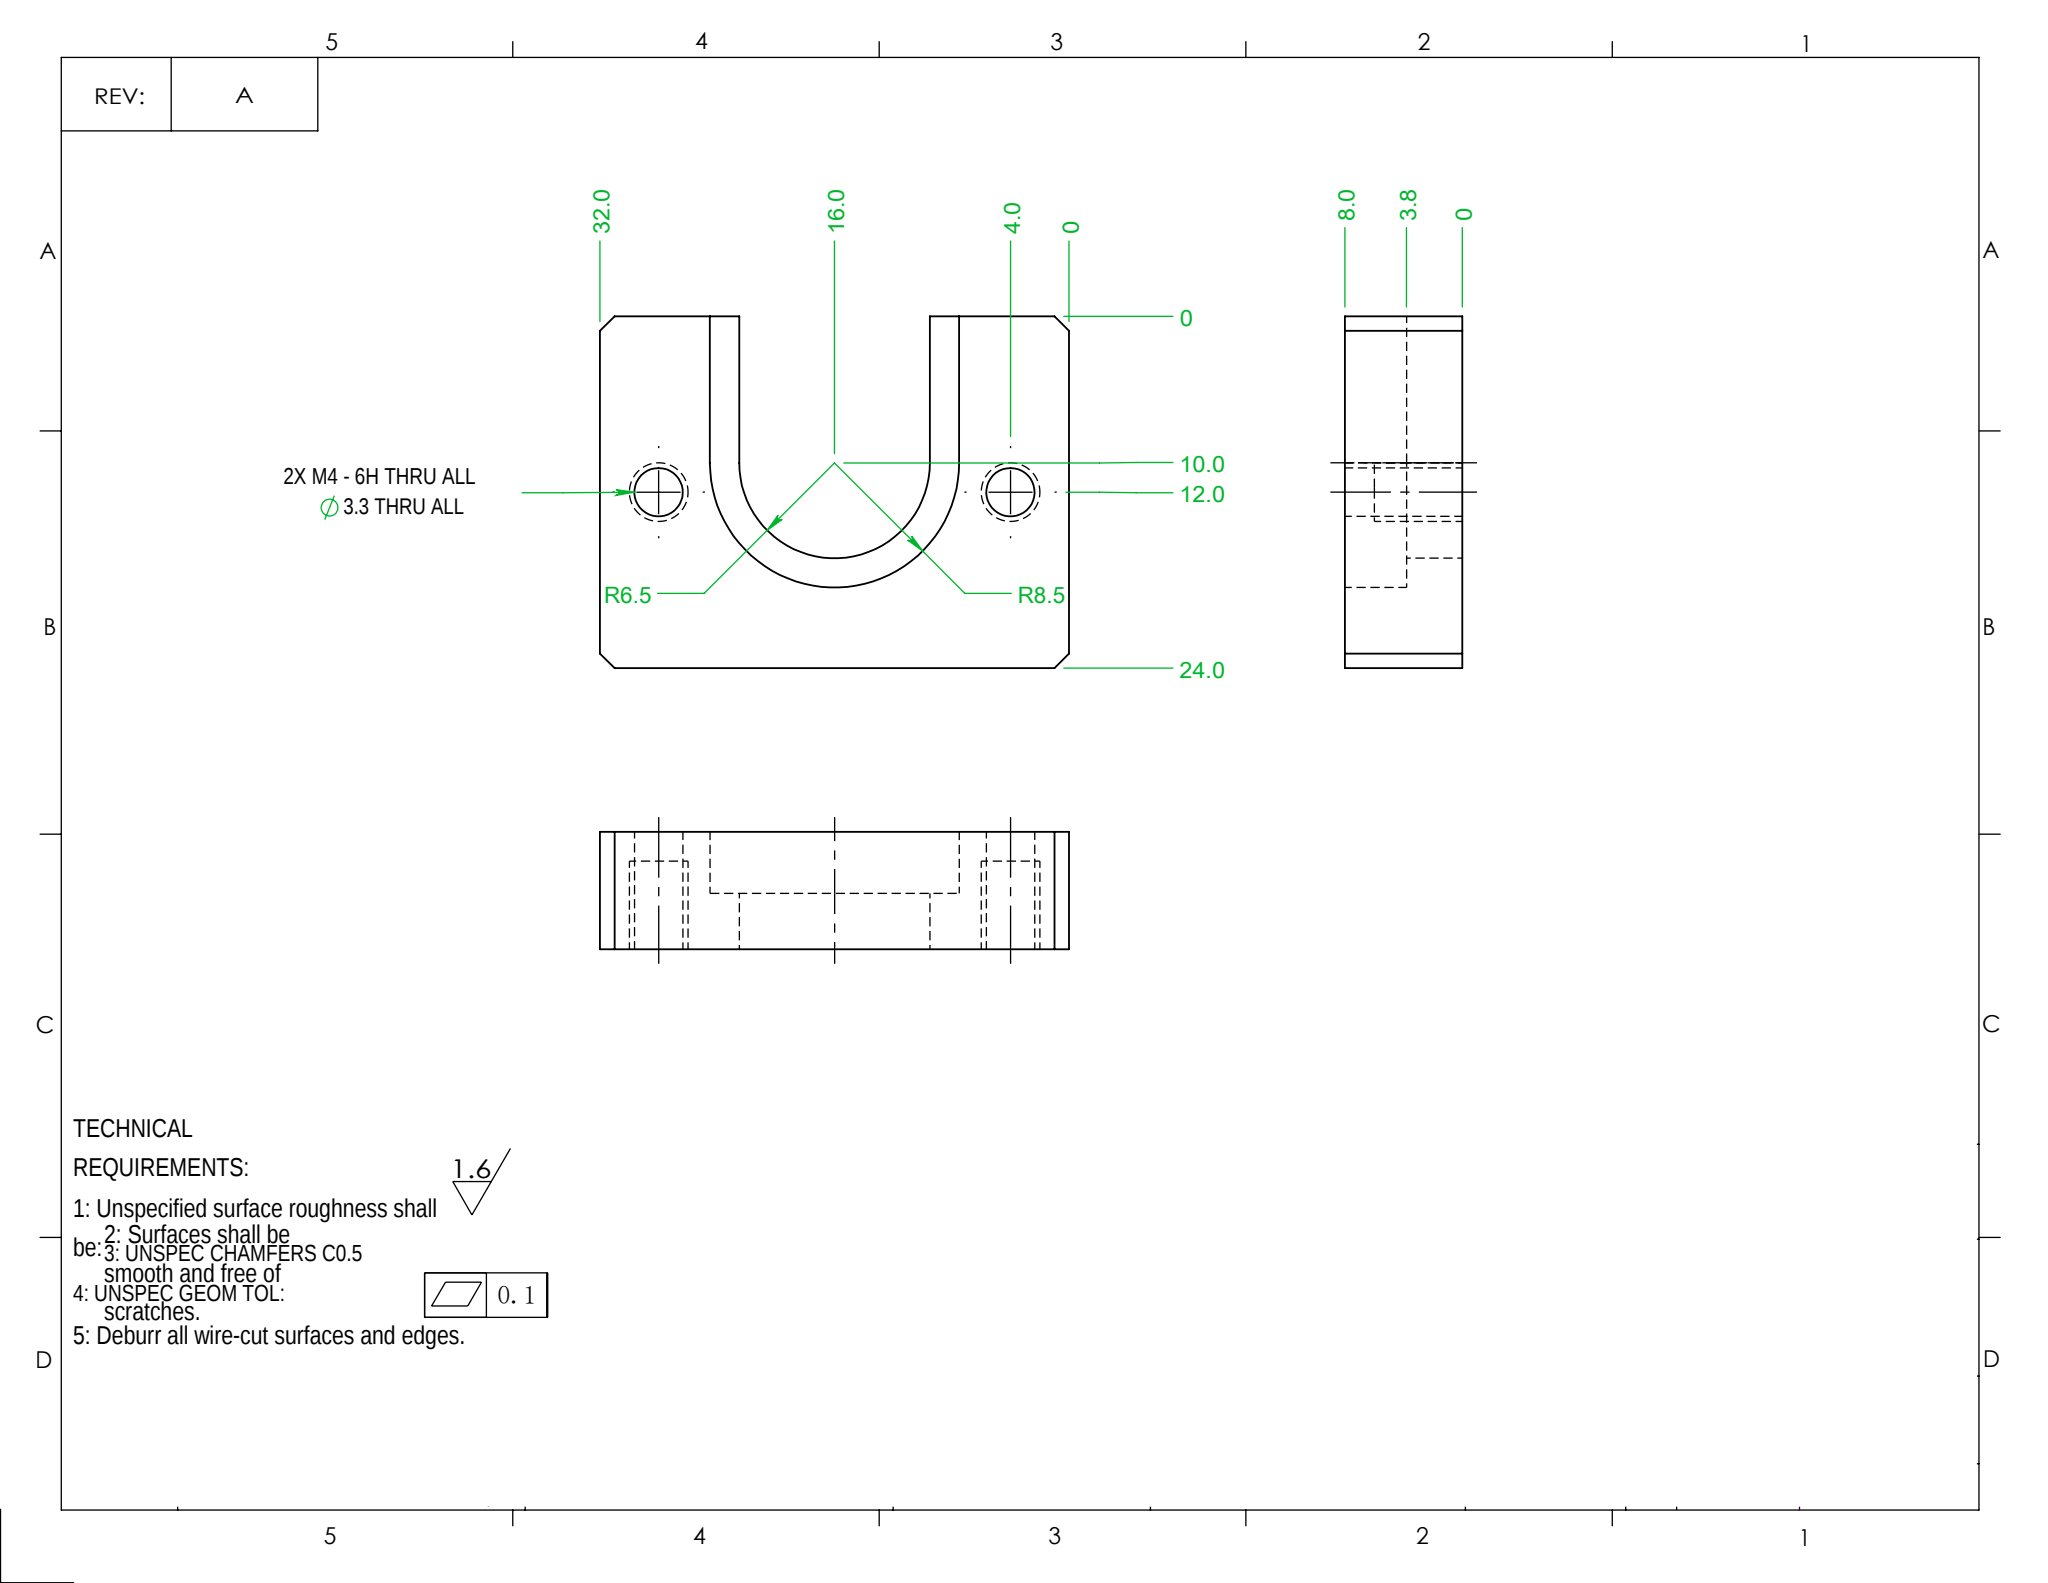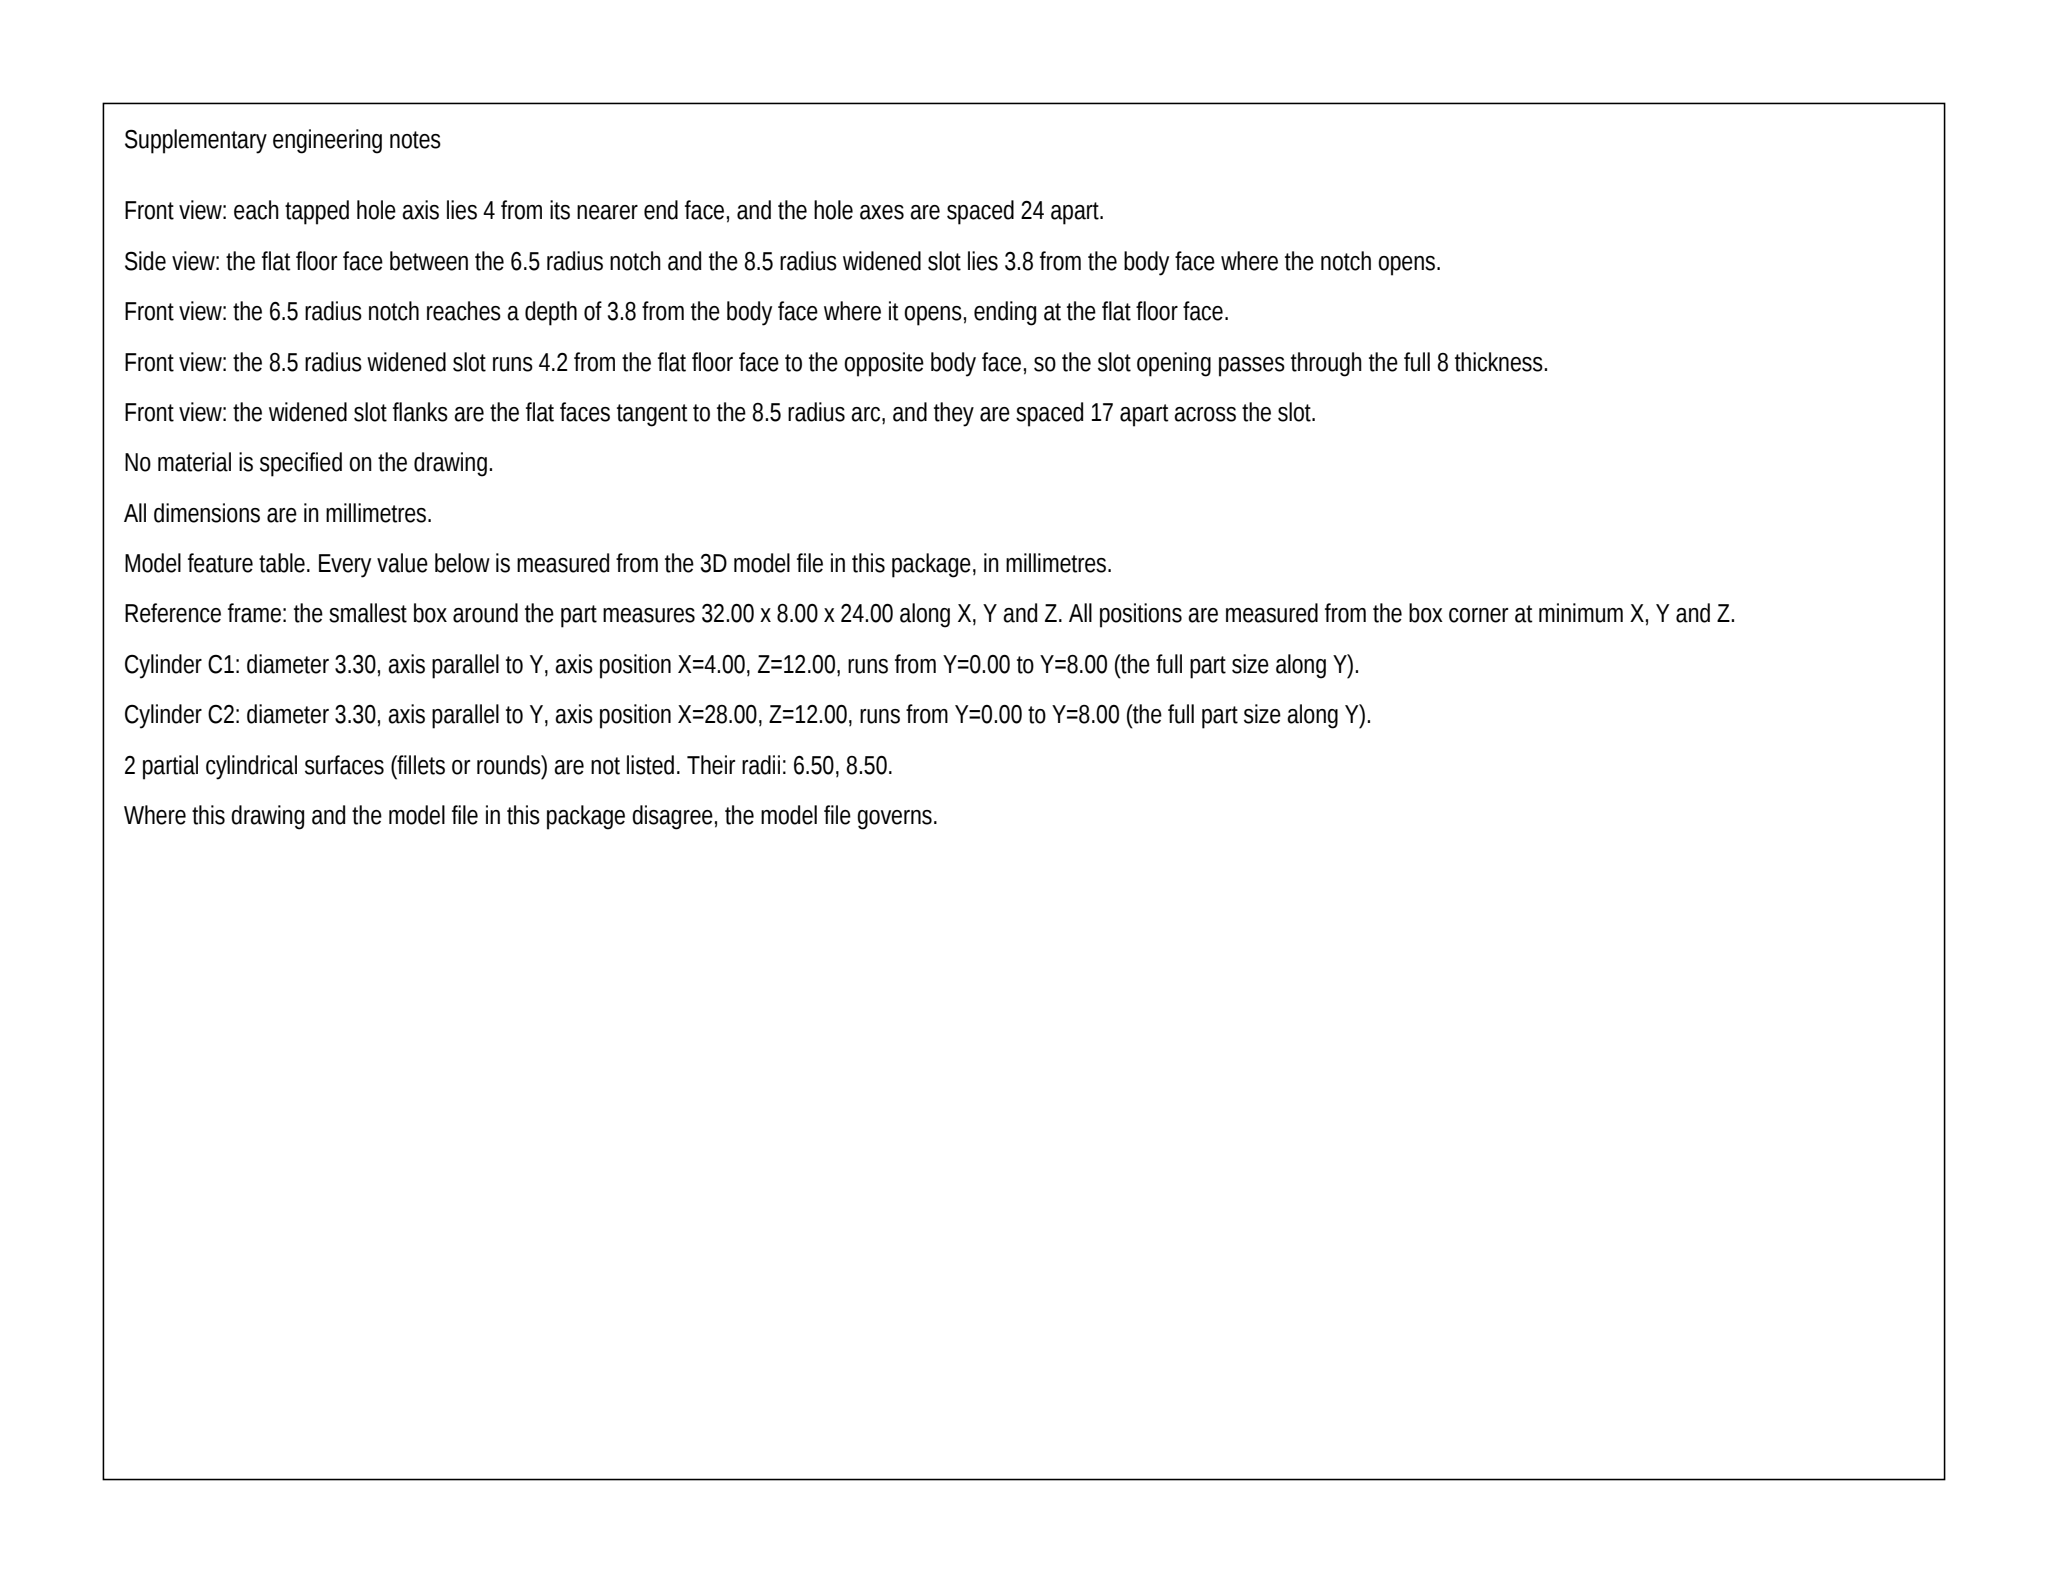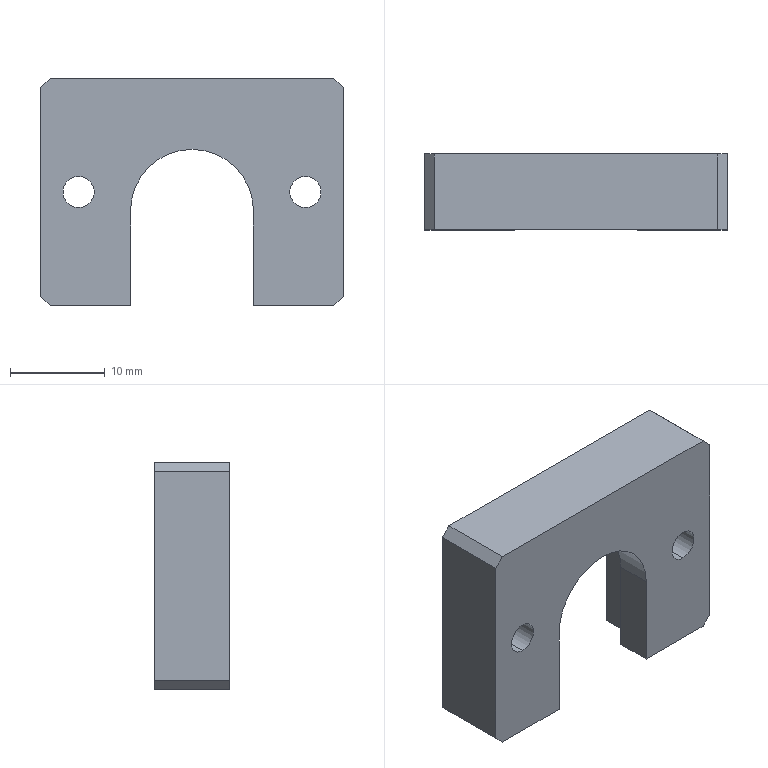Part | SolidWorks | mm | 1 solid | 24 faces | box 32 x 8 x 24 mm | volume 4054 mm3 | plane 16 | cylinder 8 | commonest cylinder face diameters 3.3 x4 13 x2 17 x2
build123d program:
from build123d import *

# Parameters (mm, degrees)
SKETCH1_W           = 32
SKETCH1_H           = 24
BOSS_EXTRUDE1_DEPTH = 8
CUT_EXTRUDE1_DEPTH  = 4.2
CUT_EXTRUDE2_DEPTH  = 41.22
CHAMFER1_SIZE       = 1
M4_TAPPED_HOLE1_D   = 3.3


with BuildPart() as part:
    # Sketch1 → Boss-Extrude1 (new body)
    with BuildSketch(Plane(origin=(0, 0, 0), x_dir=(1, 0, 0), z_dir=(0, 1, 0))):
        with Locations((16, 12)):
            Rectangle(SKETCH1_W, SKETCH1_H)
    extrude(amount=BOSS_EXTRUDE1_DEPTH)

    # Sketch2 → Cut-Extrude1 (cut)
    with BuildSketch(Plane(origin=(0, 8, 0), x_dir=(1, 0, 0), z_dir=(0, 1, 0))):
        with BuildLine():
            Line((7.5, 14), (7.5, 24))
            Line((7.5, 24), (24.5, 24))
            Line((24.5, 24), (24.5, 14))
            ThreePointArc((24.5, 14), (16, 5.5), (7.5, 14))
        make_face()
    extrude(amount=-CUT_EXTRUDE1_DEPTH, mode=Mode.SUBTRACT)

    # Sketch3 → Cut-Extrude2 (cut, through all)
    with BuildSketch(Plane(origin=(0, 3.8, 0), x_dir=(1, 0, 0), z_dir=(0, 1, 0))):
        with BuildLine():
            Line((9.5, 14), (9.5, 24))
            Line((9.5, 24), (22.5, 24))
            Line((22.5, 24), (22.5, 14))
            ThreePointArc((22.5, 14), (16, 7.5), (9.5, 14))
        make_face()
    extrude(amount=-CUT_EXTRUDE2_DEPTH, mode=Mode.SUBTRACT)

    # Chamfer1
    chamfer1_edges = [part.edges().sort_by_distance(p)[0] for p in [
        (0, 4, -24),
        (32, 4, -24),
        (32, 4, 0),
        (0, 4, 0),
    ]]
    chamfer(chamfer1_edges, length=CHAMFER1_SIZE)

    # M4 Tapped Hole1 (through all)
    with Locations(Plane(origin=(0, 0, 0), x_dir=(-1, 0, 0), z_dir=(0, -1, 0))):
        with Locations((-28, 12), (-4, 12)):
            Hole(M4_TAPPED_HOLE1_D / 2)


solid = part.part
STEP:
#1=CARTESIAN_POINT('',(28.,8.,-10.35));
#2=VERTEX_POINT('',#1);
#3=CARTESIAN_POINT('',(28.,8.,-13.65));
#4=VERTEX_POINT('',#3);
#5=CARTESIAN_POINT('',(28.,8.,-12.));
#6=DIRECTION('',(0.,-1.,0.));
#7=DIRECTION('',(0.,0.,-1.));
#8=AXIS2_PLACEMENT_3D('',#5,#6,#7);
#9=CIRCLE('',#8,1.65);
#10=EDGE_CURVE('',#2,#4,#9,.T.);
#11=ORIENTED_EDGE('',*,*,#10,.F.);
#12=CARTESIAN_POINT('',(28.,-0.,-10.35));
#13=VERTEX_POINT('',#12);
#14=CARTESIAN_POINT('',(28.,0.,-10.35));
#15=DIRECTION('',(0.,-1.,0.));
#16=VECTOR('',#15,1000.);
#17=LINE('',#14,#16);
#18=EDGE_CURVE('',#2,#13,#17,.T.);
#19=ORIENTED_EDGE('',*,*,#18,.T.);
#20=CARTESIAN_POINT('',(28.,-0.,-13.65));
#21=VERTEX_POINT('',#20);
#22=CARTESIAN_POINT('',(28.,-0.,-12.));
#23=DIRECTION('',(0.,-1.,0.));
#24=DIRECTION('',(0.,0.,-1.));
#25=AXIS2_PLACEMENT_3D('',#22,#23,#24);
#26=CIRCLE('',#25,1.65);
#27=EDGE_CURVE('',#13,#21,#26,.T.);
#28=ORIENTED_EDGE('',*,*,#27,.T.);
#29=CARTESIAN_POINT('',(28.,0.,-13.65));
#30=DIRECTION('',(0.,-1.,0.));
#31=VECTOR('',#30,1000.);
#32=LINE('',#29,#31);
#33=EDGE_CURVE('',#4,#21,#32,.T.);
#34=ORIENTED_EDGE('',*,*,#33,.F.);
#35=EDGE_LOOP('',(#11,#19,#28,#34));
#36=FACE_OUTER_BOUND('',#35,.T.);
#37=CARTESIAN_POINT('',(28.,0.,-12.));
#38=DIRECTION('',(0.,-1.,0.));
#39=DIRECTION('',(0.,0.,-1.));
#40=AXIS2_PLACEMENT_3D('',#37,#38,#39);
#41=CYLINDRICAL_SURFACE('',#40,1.65);
#42=ADVANCED_FACE('',(#36),#41,.F.);
#43=CARTESIAN_POINT('',(4.,8.,-10.35));
#44=VERTEX_POINT('',#43);
#45=CARTESIAN_POINT('',(4.,8.,-13.65));
#46=VERTEX_POINT('',#45);
#47=CARTESIAN_POINT('',(4.,8.,-12.));
#48=DIRECTION('',(0.,-1.,0.));
#49=DIRECTION('',(0.,0.,-1.));
#50=AXIS2_PLACEMENT_3D('',#47,#48,#49);
#51=CIRCLE('',#50,1.65);
#52=EDGE_CURVE('',#44,#46,#51,.T.);
#53=ORIENTED_EDGE('',*,*,#52,.F.);
#54=CARTESIAN_POINT('',(4.,-0.,-10.35));
#55=VERTEX_POINT('',#54);
#56=CARTESIAN_POINT('',(4.,0.,-10.35));
#57=DIRECTION('',(0.,-1.,0.));
#58=VECTOR('',#57,1000.);
#59=LINE('',#56,#58);
#60=EDGE_CURVE('',#44,#55,#59,.T.);
#61=ORIENTED_EDGE('',*,*,#60,.T.);
#62=CARTESIAN_POINT('',(4.,-0.,-13.65));
#63=VERTEX_POINT('',#62);
#64=CARTESIAN_POINT('',(4.,-0.,-12.));
#65=DIRECTION('',(0.,-1.,0.));
#66=DIRECTION('',(0.,0.,-1.));
#67=AXIS2_PLACEMENT_3D('',#64,#65,#66);
#68=CIRCLE('',#67,1.65);
#69=EDGE_CURVE('',#55,#63,#68,.T.);
#70=ORIENTED_EDGE('',*,*,#69,.T.);
#71=CARTESIAN_POINT('',(4.,0.,-13.65));
#72=DIRECTION('',(0.,-1.,0.));
#73=VECTOR('',#72,1000.);
#74=LINE('',#71,#73);
#75=EDGE_CURVE('',#46,#63,#74,.T.);
#76=ORIENTED_EDGE('',*,*,#75,.F.);
#77=EDGE_LOOP('',(#53,#61,#70,#76));
#78=FACE_OUTER_BOUND('',#77,.T.);
#79=CARTESIAN_POINT('',(4.,0.,-12.));
#80=DIRECTION('',(0.,-1.,0.));
#81=DIRECTION('',(0.,0.,-1.));
#82=AXIS2_PLACEMENT_3D('',#79,#80,#81);
#83=CYLINDRICAL_SURFACE('',#82,1.65);
#84=ADVANCED_FACE('',(#78),#83,.F.);
#85=CARTESIAN_POINT('',(16.,0.,-7.5));
#86=VERTEX_POINT('',#85);
#87=CARTESIAN_POINT('',(22.5,0.,-14.));
#88=VERTEX_POINT('',#87);
#89=CARTESIAN_POINT('',(16.,0.,-14.));
#90=DIRECTION('',(0.,1.,0.));
#91=DIRECTION('',(0.,0.,1.));
#92=AXIS2_PLACEMENT_3D('',#89,#90,#91);
#93=CIRCLE('',#92,6.5);
#94=EDGE_CURVE('',#86,#88,#93,.T.);
#95=ORIENTED_EDGE('',*,*,#94,.F.);
#96=CARTESIAN_POINT('',(16.,3.8,-7.5));
#97=VERTEX_POINT('',#96);
#98=CARTESIAN_POINT('',(16.,0.,-7.5));
#99=DIRECTION('',(0.,1.,0.));
#100=VECTOR('',#99,1000.);
#101=LINE('',#98,#100);
#102=EDGE_CURVE('',#86,#97,#101,.T.);
#103=ORIENTED_EDGE('',*,*,#102,.T.);
#104=CARTESIAN_POINT('',(22.5,3.8,-14.));
#105=VERTEX_POINT('',#104);
#106=CARTESIAN_POINT('',(16.,3.8,-14.));
#107=DIRECTION('',(0.,1.,0.));
#108=DIRECTION('',(0.,0.,1.));
#109=AXIS2_PLACEMENT_3D('',#106,#107,#108);
#110=CIRCLE('',#109,6.5);
#111=EDGE_CURVE('',#97,#105,#110,.T.);
#112=ORIENTED_EDGE('',*,*,#111,.T.);
#113=CARTESIAN_POINT('',(22.5,0.,-14.));
#114=DIRECTION('',(0.,1.,0.));
#115=VECTOR('',#114,1000.);
#116=LINE('',#113,#115);
#117=EDGE_CURVE('',#88,#105,#116,.T.);
#118=ORIENTED_EDGE('',*,*,#117,.F.);
#119=EDGE_LOOP('',(#95,#103,#112,#118));
#120=FACE_OUTER_BOUND('',#119,.T.);
#121=CARTESIAN_POINT('',(16.,0.,-14.));
#122=DIRECTION('',(0.,1.,0.));
#123=DIRECTION('',(0.,0.,1.));
#124=AXIS2_PLACEMENT_3D('',#121,#122,#123);
#125=CYLINDRICAL_SURFACE('',#124,6.5);
#126=ADVANCED_FACE('',(#120),#125,.F.);
#127=CARTESIAN_POINT('',(16.,3.8,-5.5));
#128=VERTEX_POINT('',#127);
#129=CARTESIAN_POINT('',(24.5,3.8,-14.));
#130=VERTEX_POINT('',#129);
#131=CARTESIAN_POINT('',(16.,3.8,-14.));
#132=DIRECTION('',(0.,1.,0.));
#133=DIRECTION('',(0.,0.,1.));
#134=AXIS2_PLACEMENT_3D('',#131,#132,#133);
#135=CIRCLE('',#134,8.5);
#136=EDGE_CURVE('',#128,#130,#135,.T.);
#137=ORIENTED_EDGE('',*,*,#136,.F.);
#138=CARTESIAN_POINT('',(16.,8.,-5.5));
#139=VERTEX_POINT('',#138);
#140=CARTESIAN_POINT('',(16.,3.8,-5.5));
#141=DIRECTION('',(0.,1.,0.));
#142=VECTOR('',#141,1000.);
#143=LINE('',#140,#142);
#144=EDGE_CURVE('',#128,#139,#143,.T.);
#145=ORIENTED_EDGE('',*,*,#144,.T.);
#146=CARTESIAN_POINT('',(24.5,8.,-14.));
#147=VERTEX_POINT('',#146);
#148=CARTESIAN_POINT('',(16.,8.,-14.));
#149=DIRECTION('',(0.,1.,0.));
#150=DIRECTION('',(0.,0.,1.));
#151=AXIS2_PLACEMENT_3D('',#148,#149,#150);
#152=CIRCLE('',#151,8.5);
#153=EDGE_CURVE('',#139,#147,#152,.T.);
#154=ORIENTED_EDGE('',*,*,#153,.T.);
#155=CARTESIAN_POINT('',(24.5,3.8,-14.));
#156=DIRECTION('',(0.,1.,0.));
#157=VECTOR('',#156,1000.);
#158=LINE('',#155,#157);
#159=EDGE_CURVE('',#130,#147,#158,.T.);
#160=ORIENTED_EDGE('',*,*,#159,.F.);
#161=EDGE_LOOP('',(#137,#145,#154,#160));
#162=FACE_OUTER_BOUND('',#161,.T.);
#163=CARTESIAN_POINT('',(16.,3.8,-14.));
#164=DIRECTION('',(0.,1.,0.));
#165=DIRECTION('',(0.,0.,1.));
#166=AXIS2_PLACEMENT_3D('',#163,#164,#165);
#167=CYLINDRICAL_SURFACE('',#166,8.5);
#168=ADVANCED_FACE('',(#162),#167,.F.);
#169=CARTESIAN_POINT('',(9.5,0.,-24.));
#170=VERTEX_POINT('',#169);
#171=CARTESIAN_POINT('',(1.,0.,-24.));
#172=VERTEX_POINT('',#171);
#173=CARTESIAN_POINT('',(0.,0.,-24.));
#174=DIRECTION('',(-1.,0.,0.));
#175=VECTOR('',#174,1000.);
#176=LINE('',#173,#175);
#177=EDGE_CURVE('',#170,#172,#176,.T.);
#178=ORIENTED_EDGE('',*,*,#177,.T.);
#179=CARTESIAN_POINT('',(1.,8.,-24.));
#180=VERTEX_POINT('',#179);
#181=CARTESIAN_POINT('',(1.,8.,-24.));
#182=DIRECTION('',(0.,1.,0.));
#183=VECTOR('',#182,1000.);
#184=LINE('',#181,#183);
#185=EDGE_CURVE('',#172,#180,#184,.T.);
#186=ORIENTED_EDGE('',*,*,#185,.T.);
#187=CARTESIAN_POINT('',(7.5,8.,-24.));
#188=VERTEX_POINT('',#187);
#189=CARTESIAN_POINT('',(0.,8.,-24.));
#190=DIRECTION('',(-1.,0.,0.));
#191=VECTOR('',#190,1000.);
#192=LINE('',#189,#191);
#193=EDGE_CURVE('',#188,#180,#192,.T.);
#194=ORIENTED_EDGE('',*,*,#193,.F.);
#195=CARTESIAN_POINT('',(7.5,3.8,-24.));
#196=VERTEX_POINT('',#195);
#197=CARTESIAN_POINT('',(7.5,3.8,-24.));
#198=DIRECTION('',(0.,1.,0.));
#199=VECTOR('',#198,1000.);
#200=LINE('',#197,#199);
#201=EDGE_CURVE('',#196,#188,#200,.T.);
#202=ORIENTED_EDGE('',*,*,#201,.F.);
#203=CARTESIAN_POINT('',(9.5,3.8,-24.));
#204=VERTEX_POINT('',#203);
#205=CARTESIAN_POINT('',(7.5,3.8,-24.));
#206=DIRECTION('',(-1.,0.,0.));
#207=VECTOR('',#206,1000.);
#208=LINE('',#205,#207);
#209=EDGE_CURVE('',#204,#196,#208,.T.);
#210=ORIENTED_EDGE('',*,*,#209,.F.);
#211=CARTESIAN_POINT('',(9.5,0.,-24.));
#212=DIRECTION('',(0.,1.,0.));
#213=VECTOR('',#212,1000.);
#214=LINE('',#211,#213);
#215=EDGE_CURVE('',#170,#204,#214,.T.);
#216=ORIENTED_EDGE('',*,*,#215,.F.);
#217=EDGE_LOOP('',(#178,#186,#194,#202,#210,#216));
#218=FACE_OUTER_BOUND('',#217,.T.);
#219=CARTESIAN_POINT('',(0.,8.,-24.));
#220=DIRECTION('',(0.,0.,1.));
#221=DIRECTION('',(1.,0.,0.));
#222=AXIS2_PLACEMENT_3D('',#219,#220,#221);
#223=PLANE('',#222);
#224=ADVANCED_FACE('',(#218),#223,.F.);
#225=CARTESIAN_POINT('',(0.,0.,-23.));
#226=VERTEX_POINT('',#225);
#227=CARTESIAN_POINT('',(0.,0.,-1.));
#228=VERTEX_POINT('',#227);
#229=CARTESIAN_POINT('',(0.,0.,0.));
#230=DIRECTION('',(-0.,0.,1.));
#231=VECTOR('',#230,1000.);
#232=LINE('',#229,#231);
#233=EDGE_CURVE('',#226,#228,#232,.T.);
#234=ORIENTED_EDGE('',*,*,#233,.T.);
#235=CARTESIAN_POINT('',(0.,8.,-1.));
#236=VERTEX_POINT('',#235);
#237=CARTESIAN_POINT('',(0.,8.,-1.));
#238=DIRECTION('',(0.,1.,0.));
#239=VECTOR('',#238,1000.);
#240=LINE('',#237,#239);
#241=EDGE_CURVE('',#228,#236,#240,.T.);
#242=ORIENTED_EDGE('',*,*,#241,.T.);
#243=CARTESIAN_POINT('',(0.,8.,-23.));
#244=VERTEX_POINT('',#243);
#245=CARTESIAN_POINT('',(0.,8.,0.));
#246=DIRECTION('',(-0.,0.,1.));
#247=VECTOR('',#246,1000.);
#248=LINE('',#245,#247);
#249=EDGE_CURVE('',#244,#236,#248,.T.);
#250=ORIENTED_EDGE('',*,*,#249,.F.);
#251=CARTESIAN_POINT('',(0.,8.,-23.));
#252=DIRECTION('',(0.,-1.,0.));
#253=VECTOR('',#252,1000.);
#254=LINE('',#251,#253);
#255=EDGE_CURVE('',#244,#226,#254,.T.);
#256=ORIENTED_EDGE('',*,*,#255,.T.);
#257=EDGE_LOOP('',(#234,#242,#250,#256));
#258=FACE_OUTER_BOUND('',#257,.T.);
#259=CARTESIAN_POINT('',(0.,8.,0.));
#260=DIRECTION('',(1.,0.,0.));
#261=DIRECTION('',(0.,0.,-1.));
#262=AXIS2_PLACEMENT_3D('',#259,#260,#261);
#263=PLANE('',#262);
#264=ADVANCED_FACE('',(#258),#263,.F.);
#265=CARTESIAN_POINT('',(1.,8.,-0.));
#266=VERTEX_POINT('',#265);
#267=CARTESIAN_POINT('',(31.,8.,-0.));
#268=VERTEX_POINT('',#267);
#269=CARTESIAN_POINT('',(0.,8.,0.));
#270=DIRECTION('',(1.,0.,0.));
#271=VECTOR('',#270,1000.);
#272=LINE('',#269,#271);
#273=EDGE_CURVE('',#266,#268,#272,.T.);
#274=ORIENTED_EDGE('',*,*,#273,.F.);
#275=CARTESIAN_POINT('',(1.,0.,-0.));
#276=VERTEX_POINT('',#275);
#277=CARTESIAN_POINT('',(1.,8.,0.));
#278=DIRECTION('',(0.,-1.,0.));
#279=VECTOR('',#278,1000.);
#280=LINE('',#277,#279);
#281=EDGE_CURVE('',#266,#276,#280,.T.);
#282=ORIENTED_EDGE('',*,*,#281,.T.);
#283=CARTESIAN_POINT('',(31.,0.,0.));
#284=VERTEX_POINT('',#283);
#285=CARTESIAN_POINT('',(0.,0.,0.));
#286=DIRECTION('',(1.,0.,0.));
#287=VECTOR('',#286,1000.);
#288=LINE('',#285,#287);
#289=EDGE_CURVE('',#276,#284,#288,.T.);
#290=ORIENTED_EDGE('',*,*,#289,.T.);
#291=CARTESIAN_POINT('',(31.,8.,0.));
#292=DIRECTION('',(0.,1.,0.));
#293=VECTOR('',#292,1000.);
#294=LINE('',#291,#293);
#295=EDGE_CURVE('',#284,#268,#294,.T.);
#296=ORIENTED_EDGE('',*,*,#295,.T.);
#297=EDGE_LOOP('',(#274,#282,#290,#296));
#298=FACE_OUTER_BOUND('',#297,.T.);
#299=CARTESIAN_POINT('',(0.,8.,0.));
#300=DIRECTION('',(0.,0.,-1.));
#301=DIRECTION('',(-1.,0.,0.));
#302=AXIS2_PLACEMENT_3D('',#299,#300,#301);
#303=PLANE('',#302);
#304=ADVANCED_FACE('',(#298),#303,.F.);
#305=CARTESIAN_POINT('',(32.,8.,-1.));
#306=VERTEX_POINT('',#305);
#307=CARTESIAN_POINT('',(32.,8.,-23.));
#308=VERTEX_POINT('',#307);
#309=CARTESIAN_POINT('',(32.,8.,0.));
#310=DIRECTION('',(-0.,0.,-1.));
#311=VECTOR('',#310,1000.);
#312=LINE('',#309,#311);
#313=EDGE_CURVE('',#306,#308,#312,.T.);
#314=ORIENTED_EDGE('',*,*,#313,.F.);
#315=CARTESIAN_POINT('',(32.,0.,-1.));
#316=VERTEX_POINT('',#315);
#317=CARTESIAN_POINT('',(32.,8.,-1.));
#318=DIRECTION('',(0.,-1.,0.));
#319=VECTOR('',#318,1000.);
#320=LINE('',#317,#319);
#321=EDGE_CURVE('',#306,#316,#320,.T.);
#322=ORIENTED_EDGE('',*,*,#321,.T.);
#323=CARTESIAN_POINT('',(32.,0.,-23.));
#324=VERTEX_POINT('',#323);
#325=CARTESIAN_POINT('',(32.,0.,0.));
#326=DIRECTION('',(-0.,0.,-1.));
#327=VECTOR('',#326,1000.);
#328=LINE('',#325,#327);
#329=EDGE_CURVE('',#316,#324,#328,.T.);
#330=ORIENTED_EDGE('',*,*,#329,.T.);
#331=CARTESIAN_POINT('',(32.,8.,-23.));
#332=DIRECTION('',(0.,1.,0.));
#333=VECTOR('',#332,1000.);
#334=LINE('',#331,#333);
#335=EDGE_CURVE('',#324,#308,#334,.T.);
#336=ORIENTED_EDGE('',*,*,#335,.T.);
#337=EDGE_LOOP('',(#314,#322,#330,#336));
#338=FACE_OUTER_BOUND('',#337,.T.);
#339=CARTESIAN_POINT('',(32.,8.,0.));
#340=DIRECTION('',(-1.,0.,0.));
#341=DIRECTION('',(0.,0.,1.));
#342=AXIS2_PLACEMENT_3D('',#339,#340,#341);
#343=PLANE('',#342);
#344=ADVANCED_FACE('',(#338),#343,.F.);
#345=CARTESIAN_POINT('',(31.,8.,-24.));
#346=VERTEX_POINT('',#345);
#347=CARTESIAN_POINT('',(24.5,8.,-24.));
#348=VERTEX_POINT('',#347);
#349=CARTESIAN_POINT('',(0.,8.,-24.));
#350=DIRECTION('',(-1.,0.,0.));
#351=VECTOR('',#350,1000.);
#352=LINE('',#349,#351);
#353=EDGE_CURVE('',#346,#348,#352,.T.);
#354=ORIENTED_EDGE('',*,*,#353,.F.);
#355=CARTESIAN_POINT('',(31.,0.,-24.));
#356=VERTEX_POINT('',#355);
#357=CARTESIAN_POINT('',(31.,8.,-24.));
#358=DIRECTION('',(0.,-1.,0.));
#359=VECTOR('',#358,1000.);
#360=LINE('',#357,#359);
#361=EDGE_CURVE('',#346,#356,#360,.T.);
#362=ORIENTED_EDGE('',*,*,#361,.T.);
#363=CARTESIAN_POINT('',(22.5,0.,-24.));
#364=VERTEX_POINT('',#363);
#365=CARTESIAN_POINT('',(0.,0.,-24.));
#366=DIRECTION('',(-1.,0.,0.));
#367=VECTOR('',#366,1000.);
#368=LINE('',#365,#367);
#369=EDGE_CURVE('',#356,#364,#368,.T.);
#370=ORIENTED_EDGE('',*,*,#369,.T.);
#371=CARTESIAN_POINT('',(22.5,3.8,-24.));
#372=VERTEX_POINT('',#371);
#373=CARTESIAN_POINT('',(22.5,0.,-24.));
#374=DIRECTION('',(0.,1.,0.));
#375=VECTOR('',#374,1000.);
#376=LINE('',#373,#375);
#377=EDGE_CURVE('',#364,#372,#376,.T.);
#378=ORIENTED_EDGE('',*,*,#377,.T.);
#379=CARTESIAN_POINT('',(24.5,3.8,-24.));
#380=VERTEX_POINT('',#379);
#381=CARTESIAN_POINT('',(7.5,3.8,-24.));
#382=DIRECTION('',(-1.,0.,0.));
#383=VECTOR('',#382,1000.);
#384=LINE('',#381,#383);
#385=EDGE_CURVE('',#380,#372,#384,.T.);
#386=ORIENTED_EDGE('',*,*,#385,.F.);
#387=CARTESIAN_POINT('',(24.5,3.8,-24.));
#388=DIRECTION('',(0.,1.,0.));
#389=VECTOR('',#388,1000.);
#390=LINE('',#387,#389);
#391=EDGE_CURVE('',#380,#348,#390,.T.);
#392=ORIENTED_EDGE('',*,*,#391,.T.);
#393=EDGE_LOOP('',(#354,#362,#370,#378,#386,#392));
#394=FACE_OUTER_BOUND('',#393,.T.);
#395=CARTESIAN_POINT('',(0.,8.,-24.));
#396=DIRECTION('',(0.,0.,1.));
#397=DIRECTION('',(1.,0.,0.));
#398=AXIS2_PLACEMENT_3D('',#395,#396,#397);
#399=PLANE('',#398);
#400=ADVANCED_FACE('',(#394),#399,.F.);
#401=CARTESIAN_POINT('',(28.,8.,-12.));
#402=DIRECTION('',(0.,-1.,0.));
#403=DIRECTION('',(0.,0.,-1.));
#404=AXIS2_PLACEMENT_3D('',#401,#402,#403);
#405=CIRCLE('',#404,1.65);
#406=EDGE_CURVE('',#4,#2,#405,.T.);
#407=ORIENTED_EDGE('',*,*,#406,.T.);
#408=ORIENTED_EDGE('',*,*,#10,.T.);
#409=EDGE_LOOP('',(#407,#408));
#410=FACE_BOUND('',#409,.T.);
#411=CARTESIAN_POINT('',(4.,8.,-12.));
#412=DIRECTION('',(0.,-1.,0.));
#413=DIRECTION('',(0.,0.,-1.));
#414=AXIS2_PLACEMENT_3D('',#411,#412,#413);
#415=CIRCLE('',#414,1.65);
#416=EDGE_CURVE('',#46,#44,#415,.T.);
#417=ORIENTED_EDGE('',*,*,#416,.T.);
#418=ORIENTED_EDGE('',*,*,#52,.T.);
#419=EDGE_LOOP('',(#417,#418));
#420=FACE_BOUND('',#419,.T.);
#421=ORIENTED_EDGE('',*,*,#249,.T.);
#422=CARTESIAN_POINT('',(1.,8.,0.));
#423=DIRECTION('',(0.7071,0.,0.7071));
#424=VECTOR('',#423,1000.);
#425=LINE('',#422,#424);
#426=EDGE_CURVE('',#236,#266,#425,.T.);
#427=ORIENTED_EDGE('',*,*,#426,.T.);
#428=ORIENTED_EDGE('',*,*,#273,.T.);
#429=CARTESIAN_POINT('',(32.,8.,-1.));
#430=DIRECTION('',(0.7071,0.,-0.7071));
#431=VECTOR('',#430,1000.);
#432=LINE('',#429,#431);
#433=EDGE_CURVE('',#268,#306,#432,.T.);
#434=ORIENTED_EDGE('',*,*,#433,.T.);
#435=ORIENTED_EDGE('',*,*,#313,.T.);
#436=CARTESIAN_POINT('',(31.,8.,-24.));
#437=DIRECTION('',(-0.7071,0.,-0.7071));
#438=VECTOR('',#437,1000.);
#439=LINE('',#436,#438);
#440=EDGE_CURVE('',#308,#346,#439,.T.);
#441=ORIENTED_EDGE('',*,*,#440,.T.);
#442=ORIENTED_EDGE('',*,*,#353,.T.);
#443=CARTESIAN_POINT('',(24.5,8.,-24.));
#444=DIRECTION('',(0.,0.,-1.));
#445=VECTOR('',#444,1000.);
#446=LINE('',#443,#445);
#447=EDGE_CURVE('',#147,#348,#446,.T.);
#448=ORIENTED_EDGE('',*,*,#447,.F.);
#449=ORIENTED_EDGE('',*,*,#153,.F.);
#450=CARTESIAN_POINT('',(7.5,8.,-14.));
#451=VERTEX_POINT('',#450);
#452=CARTESIAN_POINT('',(16.,8.,-14.));
#453=DIRECTION('',(0.,1.,0.));
#454=DIRECTION('',(0.,0.,1.));
#455=AXIS2_PLACEMENT_3D('',#452,#453,#454);
#456=CIRCLE('',#455,8.5);
#457=EDGE_CURVE('',#451,#139,#456,.T.);
#458=ORIENTED_EDGE('',*,*,#457,.F.);
#459=CARTESIAN_POINT('',(7.5,8.,-14.));
#460=DIRECTION('',(0.,0.,1.));
#461=VECTOR('',#460,1000.);
#462=LINE('',#459,#461);
#463=EDGE_CURVE('',#188,#451,#462,.T.);
#464=ORIENTED_EDGE('',*,*,#463,.F.);
#465=ORIENTED_EDGE('',*,*,#193,.T.);
#466=CARTESIAN_POINT('',(0.,8.,-23.));
#467=DIRECTION('',(-0.7071,0.,0.7071));
#468=VECTOR('',#467,1000.);
#469=LINE('',#466,#468);
#470=EDGE_CURVE('',#180,#244,#469,.T.);
#471=ORIENTED_EDGE('',*,*,#470,.T.);
#472=EDGE_LOOP('',(#421,#427,#428,#434,#435,#441,#442,#448,#449,#458,#464,#465,#471));
#473=FACE_OUTER_BOUND('',#472,.T.);
#474=CARTESIAN_POINT('',(0.,8.,0.));
#475=DIRECTION('',(0.,-1.,0.));
#476=DIRECTION('',(0.,0.,-1.));
#477=AXIS2_PLACEMENT_3D('',#474,#475,#476);
#478=PLANE('',#477);
#479=ADVANCED_FACE('',(#410,#420,#473),#478,.F.);
#480=CARTESIAN_POINT('',(28.,-0.,-12.));
#481=DIRECTION('',(0.,-1.,0.));
#482=DIRECTION('',(0.,0.,-1.));
#483=AXIS2_PLACEMENT_3D('',#480,#481,#482);
#484=CIRCLE('',#483,1.65);
#485=EDGE_CURVE('',#21,#13,#484,.T.);
#486=ORIENTED_EDGE('',*,*,#485,.F.);
#487=ORIENTED_EDGE('',*,*,#27,.F.);
#488=EDGE_LOOP('',(#486,#487));
#489=FACE_BOUND('',#488,.T.);
#490=CARTESIAN_POINT('',(4.,-0.,-12.));
#491=DIRECTION('',(0.,-1.,0.));
#492=DIRECTION('',(0.,0.,-1.));
#493=AXIS2_PLACEMENT_3D('',#490,#491,#492);
#494=CIRCLE('',#493,1.65);
#495=EDGE_CURVE('',#63,#55,#494,.T.);
#496=ORIENTED_EDGE('',*,*,#495,.F.);
#497=ORIENTED_EDGE('',*,*,#69,.F.);
#498=EDGE_LOOP('',(#496,#497));
#499=FACE_BOUND('',#498,.T.);
#500=ORIENTED_EDGE('',*,*,#289,.F.);
#501=CARTESIAN_POINT('',(0.5,0.,-0.5));
#502=DIRECTION('',(-0.7071,0.,-0.7071));
#503=VECTOR('',#502,1000.);
#504=LINE('',#501,#503);
#505=EDGE_CURVE('',#276,#228,#504,.T.);
#506=ORIENTED_EDGE('',*,*,#505,.T.);
#507=ORIENTED_EDGE('',*,*,#233,.F.);
#508=CARTESIAN_POINT('',(-11.5,0.,-11.5));
#509=DIRECTION('',(0.7071,0.,-0.7071));
#510=VECTOR('',#509,1000.);
#511=LINE('',#508,#510);
#512=EDGE_CURVE('',#226,#172,#511,.T.);
#513=ORIENTED_EDGE('',*,*,#512,.T.);
#514=ORIENTED_EDGE('',*,*,#177,.F.);
#515=CARTESIAN_POINT('',(9.5,0.,-14.));
#516=VERTEX_POINT('',#515);
#517=CARTESIAN_POINT('',(9.5,0.,-14.));
#518=DIRECTION('',(0.,0.,1.));
#519=VECTOR('',#518,1000.);
#520=LINE('',#517,#519);
#521=EDGE_CURVE('',#170,#516,#520,.T.);
#522=ORIENTED_EDGE('',*,*,#521,.T.);
#523=CARTESIAN_POINT('',(16.,0.,-14.));
#524=DIRECTION('',(0.,1.,0.));
#525=DIRECTION('',(0.,0.,1.));
#526=AXIS2_PLACEMENT_3D('',#523,#524,#525);
#527=CIRCLE('',#526,6.5);
#528=EDGE_CURVE('',#516,#86,#527,.T.);
#529=ORIENTED_EDGE('',*,*,#528,.T.);
#530=ORIENTED_EDGE('',*,*,#94,.T.);
#531=CARTESIAN_POINT('',(22.5,0.,-24.));
#532=DIRECTION('',(0.,0.,-1.));
#533=VECTOR('',#532,1000.);
#534=LINE('',#531,#533);
#535=EDGE_CURVE('',#88,#364,#534,.T.);
#536=ORIENTED_EDGE('',*,*,#535,.T.);
#537=ORIENTED_EDGE('',*,*,#369,.F.);
#538=CARTESIAN_POINT('',(27.5,0.,-27.5));
#539=DIRECTION('',(0.7071,0.,0.7071));
#540=VECTOR('',#539,1000.);
#541=LINE('',#538,#540);
#542=EDGE_CURVE('',#356,#324,#541,.T.);
#543=ORIENTED_EDGE('',*,*,#542,.T.);
#544=ORIENTED_EDGE('',*,*,#329,.F.);
#545=CARTESIAN_POINT('',(15.5,0.,15.5));
#546=DIRECTION('',(-0.7071,0.,0.7071));
#547=VECTOR('',#546,1000.);
#548=LINE('',#545,#547);
#549=EDGE_CURVE('',#316,#284,#548,.T.);
#550=ORIENTED_EDGE('',*,*,#549,.T.);
#551=EDGE_LOOP('',(#500,#506,#507,#513,#514,#522,#529,#530,#536,#537,#543,#544,#550));
#552=FACE_OUTER_BOUND('',#551,.T.);
#553=CARTESIAN_POINT('',(0.,0.,0.));
#554=DIRECTION('',(0.,-1.,0.));
#555=DIRECTION('',(0.,0.,-1.));
#556=AXIS2_PLACEMENT_3D('',#553,#554,#555);
#557=PLANE('',#556);
#558=ADVANCED_FACE('',(#489,#499,#552),#557,.T.);
#559=ORIENTED_EDGE('',*,*,#144,.F.);
#560=CARTESIAN_POINT('',(7.5,3.8,-14.));
#561=VERTEX_POINT('',#560);
#562=CARTESIAN_POINT('',(16.,3.8,-14.));
#563=DIRECTION('',(0.,1.,0.));
#564=DIRECTION('',(0.,0.,1.));
#565=AXIS2_PLACEMENT_3D('',#562,#563,#564);
#566=CIRCLE('',#565,8.5);
#567=EDGE_CURVE('',#561,#128,#566,.T.);
#568=ORIENTED_EDGE('',*,*,#567,.F.);
#569=CARTESIAN_POINT('',(7.5,3.8,-14.));
#570=DIRECTION('',(0.,1.,0.));
#571=VECTOR('',#570,1000.);
#572=LINE('',#569,#571);
#573=EDGE_CURVE('',#561,#451,#572,.T.);
#574=ORIENTED_EDGE('',*,*,#573,.T.);
#575=ORIENTED_EDGE('',*,*,#457,.T.);
#576=EDGE_LOOP('',(#559,#568,#574,#575));
#577=FACE_OUTER_BOUND('',#576,.T.);
#578=CARTESIAN_POINT('',(16.,3.8,-14.));
#579=DIRECTION('',(0.,1.,0.));
#580=DIRECTION('',(0.,0.,1.));
#581=AXIS2_PLACEMENT_3D('',#578,#579,#580);
#582=CYLINDRICAL_SURFACE('',#581,8.5);
#583=ADVANCED_FACE('',(#577),#582,.F.);
#584=ORIENTED_EDGE('',*,*,#463,.T.);
#585=ORIENTED_EDGE('',*,*,#573,.F.);
#586=CARTESIAN_POINT('',(7.5,3.8,-14.));
#587=DIRECTION('',(0.,0.,1.));
#588=VECTOR('',#587,1000.);
#589=LINE('',#586,#588);
#590=EDGE_CURVE('',#196,#561,#589,.T.);
#591=ORIENTED_EDGE('',*,*,#590,.F.);
#592=ORIENTED_EDGE('',*,*,#201,.T.);
#593=EDGE_LOOP('',(#584,#585,#591,#592));
#594=FACE_OUTER_BOUND('',#593,.T.);
#595=CARTESIAN_POINT('',(7.5,3.8,-14.));
#596=DIRECTION('',(-1.,0.,0.));
#597=DIRECTION('',(0.,0.,1.));
#598=AXIS2_PLACEMENT_3D('',#595,#596,#597);
#599=PLANE('',#598);
#600=ADVANCED_FACE('',(#594),#599,.F.);
#601=ORIENTED_EDGE('',*,*,#447,.T.);
#602=ORIENTED_EDGE('',*,*,#391,.F.);
#603=CARTESIAN_POINT('',(24.5,3.8,-24.));
#604=DIRECTION('',(0.,0.,-1.));
#605=VECTOR('',#604,1000.);
#606=LINE('',#603,#605);
#607=EDGE_CURVE('',#130,#380,#606,.T.);
#608=ORIENTED_EDGE('',*,*,#607,.F.);
#609=ORIENTED_EDGE('',*,*,#159,.T.);
#610=EDGE_LOOP('',(#601,#602,#608,#609));
#611=FACE_OUTER_BOUND('',#610,.T.);
#612=CARTESIAN_POINT('',(24.5,3.8,-24.));
#613=DIRECTION('',(1.,0.,0.));
#614=DIRECTION('',(0.,0.,-1.));
#615=AXIS2_PLACEMENT_3D('',#612,#613,#614);
#616=PLANE('',#615);
#617=ADVANCED_FACE('',(#611),#616,.F.);
#618=CARTESIAN_POINT('',(9.5,3.8,-14.));
#619=VERTEX_POINT('',#618);
#620=CARTESIAN_POINT('',(9.5,3.8,-14.));
#621=DIRECTION('',(0.,0.,1.));
#622=VECTOR('',#621,1000.);
#623=LINE('',#620,#622);
#624=EDGE_CURVE('',#204,#619,#623,.T.);
#625=ORIENTED_EDGE('',*,*,#624,.F.);
#626=ORIENTED_EDGE('',*,*,#209,.T.);
#627=ORIENTED_EDGE('',*,*,#590,.T.);
#628=ORIENTED_EDGE('',*,*,#567,.T.);
#629=ORIENTED_EDGE('',*,*,#136,.T.);
#630=ORIENTED_EDGE('',*,*,#607,.T.);
#631=ORIENTED_EDGE('',*,*,#385,.T.);
#632=CARTESIAN_POINT('',(22.5,3.8,-24.));
#633=DIRECTION('',(0.,0.,-1.));
#634=VECTOR('',#633,1000.);
#635=LINE('',#632,#634);
#636=EDGE_CURVE('',#105,#372,#635,.T.);
#637=ORIENTED_EDGE('',*,*,#636,.F.);
#638=ORIENTED_EDGE('',*,*,#111,.F.);
#639=CARTESIAN_POINT('',(16.,3.8,-14.));
#640=DIRECTION('',(0.,1.,0.));
#641=DIRECTION('',(0.,0.,1.));
#642=AXIS2_PLACEMENT_3D('',#639,#640,#641);
#643=CIRCLE('',#642,6.5);
#644=EDGE_CURVE('',#619,#97,#643,.T.);
#645=ORIENTED_EDGE('',*,*,#644,.F.);
#646=EDGE_LOOP('',(#625,#626,#627,#628,#629,#630,#631,#637,#638,#645));
#647=FACE_OUTER_BOUND('',#646,.T.);
#648=CARTESIAN_POINT('',(16.,3.8,-14.));
#649=DIRECTION('',(0.,1.,0.));
#650=DIRECTION('',(0.,0.,1.));
#651=AXIS2_PLACEMENT_3D('',#648,#649,#650);
#652=PLANE('',#651);
#653=ADVANCED_FACE('',(#647),#652,.T.);
#654=ORIENTED_EDGE('',*,*,#102,.F.);
#655=ORIENTED_EDGE('',*,*,#528,.F.);
#656=CARTESIAN_POINT('',(9.5,0.,-14.));
#657=DIRECTION('',(0.,1.,0.));
#658=VECTOR('',#657,1000.);
#659=LINE('',#656,#658);
#660=EDGE_CURVE('',#516,#619,#659,.T.);
#661=ORIENTED_EDGE('',*,*,#660,.T.);
#662=ORIENTED_EDGE('',*,*,#644,.T.);
#663=EDGE_LOOP('',(#654,#655,#661,#662));
#664=FACE_OUTER_BOUND('',#663,.T.);
#665=CARTESIAN_POINT('',(16.,0.,-14.));
#666=DIRECTION('',(0.,1.,0.));
#667=DIRECTION('',(0.,0.,1.));
#668=AXIS2_PLACEMENT_3D('',#665,#666,#667);
#669=CYLINDRICAL_SURFACE('',#668,6.5);
#670=ADVANCED_FACE('',(#664),#669,.F.);
#671=ORIENTED_EDGE('',*,*,#624,.T.);
#672=ORIENTED_EDGE('',*,*,#660,.F.);
#673=ORIENTED_EDGE('',*,*,#521,.F.);
#674=ORIENTED_EDGE('',*,*,#215,.T.);
#675=EDGE_LOOP('',(#671,#672,#673,#674));
#676=FACE_OUTER_BOUND('',#675,.T.);
#677=CARTESIAN_POINT('',(9.5,0.,-14.));
#678=DIRECTION('',(-1.,0.,0.));
#679=DIRECTION('',(0.,0.,1.));
#680=AXIS2_PLACEMENT_3D('',#677,#678,#679);
#681=PLANE('',#680);
#682=ADVANCED_FACE('',(#676),#681,.F.);
#683=ORIENTED_EDGE('',*,*,#636,.T.);
#684=ORIENTED_EDGE('',*,*,#377,.F.);
#685=ORIENTED_EDGE('',*,*,#535,.F.);
#686=ORIENTED_EDGE('',*,*,#117,.T.);
#687=EDGE_LOOP('',(#683,#684,#685,#686));
#688=FACE_OUTER_BOUND('',#687,.T.);
#689=CARTESIAN_POINT('',(22.5,0.,-24.));
#690=DIRECTION('',(1.,0.,0.));
#691=DIRECTION('',(0.,0.,-1.));
#692=AXIS2_PLACEMENT_3D('',#689,#690,#691);
#693=PLANE('',#692);
#694=ADVANCED_FACE('',(#688),#693,.F.);
#695=ORIENTED_EDGE('',*,*,#426,.F.);
#696=ORIENTED_EDGE('',*,*,#241,.F.);
#697=ORIENTED_EDGE('',*,*,#505,.F.);
#698=ORIENTED_EDGE('',*,*,#281,.F.);
#699=EDGE_LOOP('',(#695,#696,#697,#698));
#700=FACE_OUTER_BOUND('',#699,.T.);
#701=CARTESIAN_POINT('',(1.,8.,0.));
#702=DIRECTION('',(0.7071,0.,-0.7071));
#703=DIRECTION('',(0.,-1.,0.));
#704=AXIS2_PLACEMENT_3D('',#701,#702,#703);
#705=PLANE('',#704);
#706=ADVANCED_FACE('',(#700),#705,.F.);
#707=ORIENTED_EDGE('',*,*,#433,.F.);
#708=ORIENTED_EDGE('',*,*,#295,.F.);
#709=ORIENTED_EDGE('',*,*,#549,.F.);
#710=ORIENTED_EDGE('',*,*,#321,.F.);
#711=EDGE_LOOP('',(#707,#708,#709,#710));
#712=FACE_OUTER_BOUND('',#711,.T.);
#713=CARTESIAN_POINT('',(32.,8.,-1.));
#714=DIRECTION('',(-0.7071,0.,-0.7071));
#715=DIRECTION('',(0.,-1.,0.));
#716=AXIS2_PLACEMENT_3D('',#713,#714,#715);
#717=PLANE('',#716);
#718=ADVANCED_FACE('',(#712),#717,.F.);
#719=ORIENTED_EDGE('',*,*,#470,.F.);
#720=ORIENTED_EDGE('',*,*,#185,.F.);
#721=ORIENTED_EDGE('',*,*,#512,.F.);
#722=ORIENTED_EDGE('',*,*,#255,.F.);
#723=EDGE_LOOP('',(#719,#720,#721,#722));
#724=FACE_OUTER_BOUND('',#723,.T.);
#725=CARTESIAN_POINT('',(0.,8.,-23.));
#726=DIRECTION('',(0.7071,0.,0.7071));
#727=DIRECTION('',(0.,-1.,0.));
#728=AXIS2_PLACEMENT_3D('',#725,#726,#727);
#729=PLANE('',#728);
#730=ADVANCED_FACE('',(#724),#729,.F.);
#731=ORIENTED_EDGE('',*,*,#440,.F.);
#732=ORIENTED_EDGE('',*,*,#335,.F.);
#733=ORIENTED_EDGE('',*,*,#542,.F.);
#734=ORIENTED_EDGE('',*,*,#361,.F.);
#735=EDGE_LOOP('',(#731,#732,#733,#734));
#736=FACE_OUTER_BOUND('',#735,.T.);
#737=CARTESIAN_POINT('',(31.,8.,-24.));
#738=DIRECTION('',(-0.7071,0.,0.7071));
#739=DIRECTION('',(0.,-1.,0.));
#740=AXIS2_PLACEMENT_3D('',#737,#738,#739);
#741=PLANE('',#740);
#742=ADVANCED_FACE('',(#736),#741,.F.);
#743=ORIENTED_EDGE('',*,*,#60,.F.);
#744=ORIENTED_EDGE('',*,*,#416,.F.);
#745=ORIENTED_EDGE('',*,*,#75,.T.);
#746=ORIENTED_EDGE('',*,*,#495,.T.);
#747=EDGE_LOOP('',(#743,#744,#745,#746));
#748=FACE_OUTER_BOUND('',#747,.T.);
#749=CARTESIAN_POINT('',(4.,0.,-12.));
#750=DIRECTION('',(0.,-1.,0.));
#751=DIRECTION('',(0.,0.,-1.));
#752=AXIS2_PLACEMENT_3D('',#749,#750,#751);
#753=CYLINDRICAL_SURFACE('',#752,1.65);
#754=ADVANCED_FACE('',(#748),#753,.F.);
#755=ORIENTED_EDGE('',*,*,#18,.F.);
#756=ORIENTED_EDGE('',*,*,#406,.F.);
#757=ORIENTED_EDGE('',*,*,#33,.T.);
#758=ORIENTED_EDGE('',*,*,#485,.T.);
#759=EDGE_LOOP('',(#755,#756,#757,#758));
#760=FACE_OUTER_BOUND('',#759,.T.);
#761=CARTESIAN_POINT('',(28.,0.,-12.));
#762=DIRECTION('',(0.,-1.,0.));
#763=DIRECTION('',(0.,0.,-1.));
#764=AXIS2_PLACEMENT_3D('',#761,#762,#763);
#765=CYLINDRICAL_SURFACE('',#764,1.65);
#766=ADVANCED_FACE('',(#760),#765,.F.);
#767=CLOSED_SHELL('',(#42,#84,#126,#168,#224,#264,#304,#344,#400,#479,#558,#583,#600,#617,#653,#670,#682,#694,#706,#718,#730,#742,#754,#766));
#768=MANIFOLD_SOLID_BREP('',#767);
#769=CARTESIAN_POINT('',(0.,0.,0.));
#770=DIRECTION('',(0.,0.,1.));
#771=DIRECTION('',(1.,0.,0.));
#772=AXIS2_PLACEMENT_3D('',#769,#770,#771);
#773=(LENGTH_UNIT()NAMED_UNIT(*)SI_UNIT(.MILLI.,.METRE.));
#774=UNCERTAINTY_MEASURE_WITH_UNIT(LENGTH_MEASURE(0.00001),#773,'','');
#775=(NAMED_UNIT(*)PLANE_ANGLE_UNIT()SI_UNIT($,.RADIAN.));
#776=(NAMED_UNIT(*)SI_UNIT($,.STERADIAN.)SOLID_ANGLE_UNIT());
#777=(GEOMETRIC_REPRESENTATION_CONTEXT(3)GLOBAL_UNCERTAINTY_ASSIGNED_CONTEXT((#774))GLOBAL_UNIT_ASSIGNED_CONTEXT((#773,#775,#776))REPRESENTATION_CONTEXT('',''));
#778=ADVANCED_BREP_SHAPE_REPRESENTATION('',(#768,#772),#777);